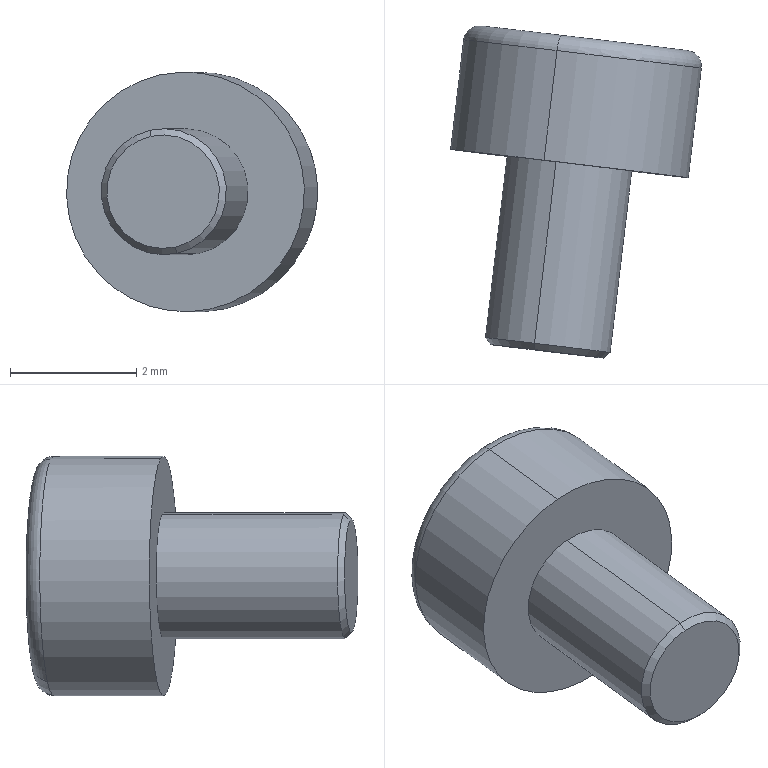Component | SolidWorks | hexagon socket head cap screws gb-2 | 1 solid | 25 faces | box 3.98 x 5.27 x 3.8 mm | volume 30 mm3 | plane 15 | cone 4 | cylinder 4 | torus 2 | commonest cylinder face diameters 2 x2 3.8 x2
STEP:
#1=CARTESIAN_POINT('',(-0.1815,3.084,0.2292));
#2=VERTEX_POINT('',#1);
#3=CARTESIAN_POINT('',(-0.1966,3.086,0.2984));
#4=VERTEX_POINT('',#3);
#5=CARTESIAN_POINT('',(-0.189,3.085,0.2638));
#6=DIRECTION('',(-0.1183,-0.993,0.001159));
#7=DIRECTION('',(0.2126,-0.02647,-0.9768));
#8=AXIS2_PLACEMENT_3D('',#5,#6,#7);
#9=CIRCLE('',#8,0.03543);
#10=EDGE_CURVE('',#2,#4,#9,.T.);
#11=ORIENTED_EDGE('',*,*,#10,.F.);
#12=CARTESIAN_POINT('',(-0.1802,3.088,0.2254));
#13=VERTEX_POINT('',#12);
#14=CARTESIAN_POINT('',(-0.1815,3.084,0.2292));
#15=DIRECTION('',(0.234,0.6834,-0.6915));
#16=VECTOR('',#15,39.37);
#17=LINE('',#14,#16);
#18=EDGE_CURVE('',#2,#13,#17,.T.);
#19=ORIENTED_EDGE('',*,*,#18,.T.);
#20=CARTESIAN_POINT('',(-0.1969,3.09,0.3023));
#21=VERTEX_POINT('',#20);
#22=CARTESIAN_POINT('',(-0.1886,3.089,0.2638));
#23=DIRECTION('',(0.1183,0.993,-0.001159));
#24=DIRECTION('',(0.2126,-0.02647,-0.9768));
#25=AXIS2_PLACEMENT_3D('',#22,#23,#24);
#26=CIRCLE('',#25,0.03937);
#27=EDGE_CURVE('',#21,#13,#26,.T.);
#28=ORIENTED_EDGE('',*,*,#27,.F.);
#29=CARTESIAN_POINT('',(-0.1966,3.086,0.2984));
#30=DIRECTION('',(-0.06668,0.7209,0.6899));
#31=VECTOR('',#30,39.37);
#32=LINE('',#29,#31);
#33=EDGE_CURVE('',#4,#21,#32,.T.);
#34=ORIENTED_EDGE('',*,*,#33,.F.);
#35=EDGE_LOOP('',(#11,#19,#28,#34));
#36=FACE_OUTER_BOUND('',#35,.T.);
#37=CARTESIAN_POINT('',(-0.189,3.085,0.2638));
#38=DIRECTION('',(0.1183,0.993,-0.001159));
#39=DIRECTION('',(-0.2126,0.02647,0.9768));
#40=AXIS2_PLACEMENT_3D('',#37,#38,#39);
#41=CONICAL_SURFACE('',#40,0.03543,0.7854);
#42=ADVANCED_FACE('',(#36),#41,.T.);
#43=CARTESIAN_POINT('',(-0.1796,3.283,0.3271));
#44=VERTEX_POINT('',#43);
#45=CARTESIAN_POINT('',(-0.1519,3.279,0.2002));
#46=VERTEX_POINT('',#45);
#47=CARTESIAN_POINT('',(-0.1658,3.281,0.2636));
#48=DIRECTION('',(0.1183,0.993,-0.001159));
#49=DIRECTION('',(0.2126,-0.02647,-0.9768));
#50=AXIS2_PLACEMENT_3D('',#47,#48,#49);
#51=CIRCLE('',#50,0.06496);
#52=EDGE_CURVE('',#44,#46,#51,.T.);
#53=ORIENTED_EDGE('',*,*,#52,.F.);
#54=CARTESIAN_POINT('',(-0.1828,3.273,0.3367));
#55=VERTEX_POINT('',#54);
#56=CARTESIAN_POINT('',(-0.1807,3.273,0.3271));
#57=DIRECTION('',(0.9699,-0.1153,0.2143));
#58=DIRECTION('',(0.2157,0.,-0.9765));
#59=AXIS2_PLACEMENT_3D('',#56,#57,#58);
#60=CIRCLE('',#59,0.009843);
#61=EDGE_CURVE('',#44,#55,#60,.T.);
#62=ORIENTED_EDGE('',*,*,#61,.T.);
#63=CARTESIAN_POINT('',(-0.151,3.269,0.1906));
#64=VERTEX_POINT('',#63);
#65=CARTESIAN_POINT('',(-0.1669,3.271,0.2636));
#66=DIRECTION('',(-0.1183,-0.993,0.001159));
#67=DIRECTION('',(0.2126,-0.02647,-0.9768));
#68=AXIS2_PLACEMENT_3D('',#65,#66,#67);
#69=CIRCLE('',#68,0.0748);
#70=EDGE_CURVE('',#64,#55,#69,.T.);
#71=ORIENTED_EDGE('',*,*,#70,.F.);
#72=CARTESIAN_POINT('',(-0.1531,3.269,0.2002));
#73=DIRECTION('',(-0.9699,0.1153,-0.2143));
#74=DIRECTION('',(-0.2157,0.,0.9765));
#75=AXIS2_PLACEMENT_3D('',#72,#73,#74);
#76=CIRCLE('',#75,0.009843);
#77=EDGE_CURVE('',#46,#64,#76,.T.);
#78=ORIENTED_EDGE('',*,*,#77,.F.);
#79=EDGE_LOOP('',(#53,#62,#71,#78));
#80=FACE_OUTER_BOUND('',#79,.T.);
#81=CARTESIAN_POINT('',(-0.1669,3.271,0.2636));
#82=DIRECTION('',(-0.1183,-0.993,0.001159));
#83=DIRECTION('',(0.2126,-0.02647,-0.9768));
#84=AXIS2_PLACEMENT_3D('',#81,#82,#83);
#85=TOROIDAL_SURFACE('',#84,0.06496,0.009843);
#86=ADVANCED_FACE('',(#80),#85,.T.);
#87=CARTESIAN_POINT('',(-0.1724,3.225,0.2637));
#88=VERTEX_POINT('',#87);
#89=CARTESIAN_POINT('',(-0.1767,3.243,0.2925));
#90=VERTEX_POINT('',#89);
#91=CARTESIAN_POINT('',(-0.1767,3.243,0.2925));
#92=DIRECTION('',(-0.125,0.5194,0.8453));
#93=VECTOR('',#92,39.37);
#94=LINE('',#91,#93);
#95=EDGE_CURVE('',#88,#90,#94,.T.);
#96=ORIENTED_EDGE('',*,*,#95,.F.);
#97=CARTESIAN_POINT('',(-0.1641,3.241,0.2348));
#98=VERTEX_POINT('',#97);
#99=CARTESIAN_POINT('',(-0.1641,3.241,0.2348));
#100=DIRECTION('',(0.2433,0.4736,-0.8465));
#101=VECTOR('',#100,39.37);
#102=LINE('',#99,#101);
#103=EDGE_CURVE('',#88,#98,#102,.T.);
#104=ORIENTED_EDGE('',*,*,#103,.T.);
#105=CARTESIAN_POINT('',(-0.1793,3.243,0.2355));
#106=VERTEX_POINT('',#105);
#107=CARTESIAN_POINT('',(-0.1704,3.242,0.2637));
#108=DIRECTION('',(-0.1183,-0.993,0.001159));
#109=DIRECTION('',(-0.2126,0.02647,0.9768));
#110=AXIS2_PLACEMENT_3D('',#107,#108,#109);
#111=CIRCLE('',#110,0.02953);
#112=EDGE_CURVE('',#106,#98,#111,.T.);
#113=ORIENTED_EDGE('',*,*,#112,.F.);
#114=CARTESIAN_POINT('',(-0.1991,3.245,0.2573));
#115=VERTEX_POINT('',#114);
#116=CARTESIAN_POINT('',(-0.1704,3.242,0.2637));
#117=DIRECTION('',(-0.1183,-0.993,0.001159));
#118=DIRECTION('',(-0.2126,0.02647,0.9768));
#119=AXIS2_PLACEMENT_3D('',#116,#117,#118);
#120=CIRCLE('',#119,0.02953);
#121=EDGE_CURVE('',#115,#106,#120,.T.);
#122=ORIENTED_EDGE('',*,*,#121,.F.);
#123=CARTESIAN_POINT('',(-0.1902,3.244,0.2855));
#124=VERTEX_POINT('',#123);
#125=CARTESIAN_POINT('',(-0.1704,3.242,0.2637));
#126=DIRECTION('',(-0.1183,-0.993,0.001159));
#127=DIRECTION('',(-0.2126,0.02647,0.9768));
#128=AXIS2_PLACEMENT_3D('',#125,#126,#127);
#129=CIRCLE('',#128,0.02953);
#130=EDGE_CURVE('',#124,#115,#129,.T.);
#131=ORIENTED_EDGE('',*,*,#130,.F.);
#132=CARTESIAN_POINT('',(-0.1704,3.242,0.2637));
#133=DIRECTION('',(-0.1183,-0.993,0.001159));
#134=DIRECTION('',(-0.2126,0.02647,0.9768));
#135=AXIS2_PLACEMENT_3D('',#132,#133,#134);
#136=CIRCLE('',#135,0.02953);
#137=EDGE_CURVE('',#90,#124,#136,.T.);
#138=ORIENTED_EDGE('',*,*,#137,.F.);
#139=EDGE_LOOP('',(#96,#104,#113,#122,#131,#138));
#140=FACE_OUTER_BOUND('',#139,.T.);
#141=CARTESIAN_POINT('',(-0.1704,3.242,0.2637));
#142=DIRECTION('',(0.1183,0.993,-0.001159));
#143=DIRECTION('',(-0.2126,0.02647,0.9768));
#144=AXIS2_PLACEMENT_3D('',#141,#142,#143);
#145=CONICAL_SURFACE('',#144,0.02953,1.047);
#146=ADVANCED_FACE('',(#140),#145,.F.);
#147=ORIENTED_EDGE('',*,*,#27,.T.);
#148=CARTESIAN_POINT('',(-0.1667,3.202,0.2252));
#149=VERTEX_POINT('',#148);
#150=CARTESIAN_POINT('',(-0.1807,3.084,0.2254));
#151=DIRECTION('',(0.1183,0.993,-0.001159));
#152=VECTOR('',#151,39.37);
#153=LINE('',#150,#152);
#154=EDGE_CURVE('',#13,#149,#153,.T.);
#155=ORIENTED_EDGE('',*,*,#154,.T.);
#156=CARTESIAN_POINT('',(-0.1834,3.204,0.3022));
#157=VERTEX_POINT('',#156);
#158=CARTESIAN_POINT('',(-0.1751,3.203,0.2637));
#159=DIRECTION('',(-0.1183,-0.993,0.001159));
#160=DIRECTION('',(0.2126,-0.02647,-0.9768));
#161=AXIS2_PLACEMENT_3D('',#158,#159,#160);
#162=CIRCLE('',#161,0.03937);
#163=EDGE_CURVE('',#149,#157,#162,.T.);
#164=ORIENTED_EDGE('',*,*,#163,.T.);
#165=CARTESIAN_POINT('',(-0.1974,3.086,0.3023));
#166=DIRECTION('',(0.1183,0.993,-0.001159));
#167=VECTOR('',#166,39.37);
#168=LINE('',#165,#167);
#169=EDGE_CURVE('',#21,#157,#168,.T.);
#170=ORIENTED_EDGE('',*,*,#169,.F.);
#171=EDGE_LOOP('',(#147,#155,#164,#170));
#172=FACE_OUTER_BOUND('',#171,.T.);
#173=CARTESIAN_POINT('',(-0.189,3.085,0.2638));
#174=DIRECTION('',(0.1183,0.993,-0.001159));
#175=DIRECTION('',(-0.2126,0.02647,0.9768));
#176=AXIS2_PLACEMENT_3D('',#173,#174,#175);
#177=CYLINDRICAL_SURFACE('',#176,0.03937);
#178=ADVANCED_FACE('',(#172),#177,.T.);
#179=CARTESIAN_POINT('',(-0.1592,3.201,0.1906));
#180=VERTEX_POINT('',#179);
#181=CARTESIAN_POINT('',(-0.191,3.205,0.3368));
#182=VERTEX_POINT('',#181);
#183=CARTESIAN_POINT('',(-0.1751,3.203,0.2637));
#184=DIRECTION('',(-0.1183,-0.993,0.001159));
#185=DIRECTION('',(0.2126,-0.02647,-0.9768));
#186=AXIS2_PLACEMENT_3D('',#183,#184,#185);
#187=CIRCLE('',#186,0.0748);
#188=EDGE_CURVE('',#180,#182,#187,.T.);
#189=ORIENTED_EDGE('',*,*,#188,.F.);
#190=CARTESIAN_POINT('',(-0.1592,3.201,0.1906));
#191=DIRECTION('',(0.1183,0.993,-0.001159));
#192=VECTOR('',#191,39.37);
#193=LINE('',#190,#192);
#194=EDGE_CURVE('',#180,#64,#193,.T.);
#195=ORIENTED_EDGE('',*,*,#194,.T.);
#196=ORIENTED_EDGE('',*,*,#70,.T.);
#197=CARTESIAN_POINT('',(-0.191,3.205,0.3368));
#198=DIRECTION('',(0.1183,0.993,-0.001159));
#199=VECTOR('',#198,39.37);
#200=LINE('',#197,#199);
#201=EDGE_CURVE('',#182,#55,#200,.T.);
#202=ORIENTED_EDGE('',*,*,#201,.F.);
#203=EDGE_LOOP('',(#189,#195,#196,#202));
#204=FACE_OUTER_BOUND('',#203,.T.);
#205=CARTESIAN_POINT('',(-0.1751,3.203,0.2637));
#206=DIRECTION('',(0.1183,0.993,-0.001159));
#207=DIRECTION('',(-0.2126,0.02647,0.9768));
#208=AXIS2_PLACEMENT_3D('',#205,#206,#207);
#209=CYLINDRICAL_SURFACE('',#208,0.0748);
#210=ADVANCED_FACE('',(#204),#209,.T.);
#211=CARTESIAN_POINT('',(-0.2027,3.246,0.274));
#212=VERTEX_POINT('',#211);
#213=CARTESIAN_POINT('',(-0.1777,3.243,0.297));
#214=DIRECTION('',(-0.7337,0.08664,-0.6739));
#215=VECTOR('',#214,39.37);
#216=LINE('',#213,#215);
#217=EDGE_CURVE('',#124,#212,#216,.T.);
#218=ORIENTED_EDGE('',*,*,#217,.F.);
#219=ORIENTED_EDGE('',*,*,#130,.T.);
#220=CARTESIAN_POINT('',(-0.2027,3.246,0.274));
#221=DIRECTION('',(0.2126,-0.02647,-0.9768));
#222=VECTOR('',#221,39.37);
#223=LINE('',#220,#222);
#224=EDGE_CURVE('',#212,#115,#223,.T.);
#225=ORIENTED_EDGE('',*,*,#224,.F.);
#226=EDGE_LOOP('',(#218,#219,#225));
#227=FACE_OUTER_BOUND('',#226,.T.);
#228=CARTESIAN_POINT('',(-0.2277,3.249,0.251));
#229=DIRECTION('',(0.1183,0.993,-0.001159));
#230=DIRECTION('',(-0.2126,0.02647,0.9768));
#231=AXIS2_PLACEMENT_3D('',#228,#229,#230);
#232=PLANE('',#231);
#233=ADVANCED_FACE('',(#227),#232,.T.);
#234=CARTESIAN_POINT('',(-0.1954,3.245,0.2407));
#235=VERTEX_POINT('',#234);
#236=CARTESIAN_POINT('',(-0.2027,3.246,0.274));
#237=DIRECTION('',(0.2126,-0.02647,-0.9768));
#238=VECTOR('',#237,39.37);
#239=LINE('',#236,#238);
#240=EDGE_CURVE('',#115,#235,#239,.T.);
#241=ORIENTED_EDGE('',*,*,#240,.F.);
#242=ORIENTED_EDGE('',*,*,#121,.T.);
#243=CARTESIAN_POINT('',(-0.1954,3.245,0.2407));
#244=DIRECTION('',(0.9463,-0.1131,-0.3028));
#245=VECTOR('',#244,39.37);
#246=LINE('',#243,#245);
#247=EDGE_CURVE('',#235,#106,#246,.T.);
#248=ORIENTED_EDGE('',*,*,#247,.F.);
#249=EDGE_LOOP('',(#241,#242,#248));
#250=FACE_OUTER_BOUND('',#249,.T.);
#251=CARTESIAN_POINT('',(-0.2277,3.249,0.251));
#252=DIRECTION('',(0.1183,0.993,-0.001159));
#253=DIRECTION('',(-0.2126,0.02647,0.9768));
#254=AXIS2_PLACEMENT_3D('',#251,#252,#253);
#255=PLANE('',#254);
#256=ADVANCED_FACE('',(#250),#255,.T.);
#257=CARTESIAN_POINT('',(-0.1632,3.241,0.2304));
#258=VERTEX_POINT('',#257);
#259=CARTESIAN_POINT('',(-0.1954,3.245,0.2407));
#260=DIRECTION('',(0.9463,-0.1131,-0.3028));
#261=VECTOR('',#260,39.37);
#262=LINE('',#259,#261);
#263=EDGE_CURVE('',#106,#258,#262,.T.);
#264=ORIENTED_EDGE('',*,*,#263,.F.);
#265=ORIENTED_EDGE('',*,*,#112,.T.);
#266=CARTESIAN_POINT('',(-0.1507,3.239,0.2418));
#267=VERTEX_POINT('',#266);
#268=CARTESIAN_POINT('',(-0.1704,3.242,0.2637));
#269=DIRECTION('',(-0.1183,-0.993,0.001159));
#270=DIRECTION('',(-0.2126,0.02647,0.9768));
#271=AXIS2_PLACEMENT_3D('',#268,#269,#270);
#272=CIRCLE('',#271,0.02953);
#273=EDGE_CURVE('',#98,#267,#272,.T.);
#274=ORIENTED_EDGE('',*,*,#273,.T.);
#275=CARTESIAN_POINT('',(-0.1632,3.241,0.2304));
#276=DIRECTION('',(0.7337,-0.08664,0.6739));
#277=VECTOR('',#276,39.37);
#278=LINE('',#275,#277);
#279=EDGE_CURVE('',#258,#267,#278,.T.);
#280=ORIENTED_EDGE('',*,*,#279,.F.);
#281=EDGE_LOOP('',(#264,#265,#274,#280));
#282=FACE_OUTER_BOUND('',#281,.T.);
#283=CARTESIAN_POINT('',(-0.2277,3.249,0.251));
#284=DIRECTION('',(0.1183,0.993,-0.001159));
#285=DIRECTION('',(-0.2126,0.02647,0.9768));
#286=AXIS2_PLACEMENT_3D('',#283,#284,#285);
#287=PLANE('',#286);
#288=ADVANCED_FACE('',(#282),#287,.T.);
#289=CARTESIAN_POINT('',(-0.1381,3.238,0.2533));
#290=VERTEX_POINT('',#289);
#291=CARTESIAN_POINT('',(-0.1632,3.241,0.2304));
#292=DIRECTION('',(0.7337,-0.08664,0.6739));
#293=VECTOR('',#292,39.37);
#294=LINE('',#291,#293);
#295=EDGE_CURVE('',#267,#290,#294,.T.);
#296=ORIENTED_EDGE('',*,*,#295,.F.);
#297=CARTESIAN_POINT('',(-0.1418,3.238,0.27));
#298=VERTEX_POINT('',#297);
#299=CARTESIAN_POINT('',(-0.1704,3.242,0.2637));
#300=DIRECTION('',(-0.1183,-0.993,0.001159));
#301=DIRECTION('',(0.2126,-0.02647,-0.9768));
#302=AXIS2_PLACEMENT_3D('',#299,#300,#301);
#303=CIRCLE('',#302,0.02953);
#304=EDGE_CURVE('',#267,#298,#303,.T.);
#305=ORIENTED_EDGE('',*,*,#304,.T.);
#306=CARTESIAN_POINT('',(-0.1381,3.238,0.2533));
#307=DIRECTION('',(-0.2126,0.02647,0.9768));
#308=VECTOR('',#307,39.37);
#309=LINE('',#306,#308);
#310=EDGE_CURVE('',#290,#298,#309,.T.);
#311=ORIENTED_EDGE('',*,*,#310,.F.);
#312=EDGE_LOOP('',(#296,#305,#311));
#313=FACE_OUTER_BOUND('',#312,.T.);
#314=CARTESIAN_POINT('',(-0.2277,3.249,0.251));
#315=DIRECTION('',(0.1183,0.993,-0.001159));
#316=DIRECTION('',(-0.2126,0.02647,0.9768));
#317=AXIS2_PLACEMENT_3D('',#314,#315,#316);
#318=PLANE('',#317);
#319=ADVANCED_FACE('',(#313),#318,.T.);
#320=CARTESIAN_POINT('',(-0.1454,3.239,0.2866));
#321=VERTEX_POINT('',#320);
#322=CARTESIAN_POINT('',(-0.1381,3.238,0.2533));
#323=DIRECTION('',(-0.2126,0.02647,0.9768));
#324=VECTOR('',#323,39.37);
#325=LINE('',#322,#324);
#326=EDGE_CURVE('',#298,#321,#325,.T.);
#327=ORIENTED_EDGE('',*,*,#326,.F.);
#328=CARTESIAN_POINT('',(-0.1615,3.241,0.2918));
#329=VERTEX_POINT('',#328);
#330=CARTESIAN_POINT('',(-0.1704,3.242,0.2637));
#331=DIRECTION('',(-0.1183,-0.993,0.001159));
#332=DIRECTION('',(-0.2126,0.02647,0.9768));
#333=AXIS2_PLACEMENT_3D('',#330,#331,#332);
#334=CIRCLE('',#333,0.02953);
#335=EDGE_CURVE('',#298,#329,#334,.T.);
#336=ORIENTED_EDGE('',*,*,#335,.T.);
#337=CARTESIAN_POINT('',(-0.1454,3.239,0.2866));
#338=DIRECTION('',(-0.9463,0.1131,0.3028));
#339=VECTOR('',#338,39.37);
#340=LINE('',#337,#339);
#341=EDGE_CURVE('',#321,#329,#340,.T.);
#342=ORIENTED_EDGE('',*,*,#341,.F.);
#343=EDGE_LOOP('',(#327,#336,#342));
#344=FACE_OUTER_BOUND('',#343,.T.);
#345=CARTESIAN_POINT('',(-0.2277,3.249,0.251));
#346=DIRECTION('',(0.1183,0.993,-0.001159));
#347=DIRECTION('',(-0.2126,0.02647,0.9768));
#348=AXIS2_PLACEMENT_3D('',#345,#346,#347);
#349=PLANE('',#348);
#350=ADVANCED_FACE('',(#344),#349,.T.);
#351=CARTESIAN_POINT('',(-0.1777,3.243,0.297));
#352=VERTEX_POINT('',#351);
#353=CARTESIAN_POINT('',(-0.1454,3.239,0.2866));
#354=DIRECTION('',(-0.9463,0.1131,0.3028));
#355=VECTOR('',#354,39.37);
#356=LINE('',#353,#355);
#357=EDGE_CURVE('',#329,#352,#356,.T.);
#358=ORIENTED_EDGE('',*,*,#357,.F.);
#359=CARTESIAN_POINT('',(-0.1704,3.242,0.2637));
#360=DIRECTION('',(-0.1183,-0.993,0.001159));
#361=DIRECTION('',(-0.2126,0.02647,0.9768));
#362=AXIS2_PLACEMENT_3D('',#359,#360,#361);
#363=CIRCLE('',#362,0.02953);
#364=EDGE_CURVE('',#329,#90,#363,.T.);
#365=ORIENTED_EDGE('',*,*,#364,.T.);
#366=ORIENTED_EDGE('',*,*,#137,.T.);
#367=CARTESIAN_POINT('',(-0.1777,3.243,0.297));
#368=DIRECTION('',(-0.7337,0.08664,-0.6739));
#369=VECTOR('',#368,39.37);
#370=LINE('',#367,#369);
#371=EDGE_CURVE('',#352,#124,#370,.T.);
#372=ORIENTED_EDGE('',*,*,#371,.F.);
#373=EDGE_LOOP('',(#358,#365,#366,#372));
#374=FACE_OUTER_BOUND('',#373,.T.);
#375=CARTESIAN_POINT('',(-0.2277,3.249,0.251));
#376=DIRECTION('',(0.1183,0.993,-0.001159));
#377=DIRECTION('',(-0.2126,0.02647,0.9768));
#378=AXIS2_PLACEMENT_3D('',#375,#376,#377);
#379=PLANE('',#378);
#380=ADVANCED_FACE('',(#374),#379,.T.);
#381=CARTESIAN_POINT('',(-0.1658,3.281,0.2636));
#382=DIRECTION('',(0.1183,0.993,-0.001159));
#383=DIRECTION('',(0.2126,-0.02647,-0.9768));
#384=AXIS2_PLACEMENT_3D('',#381,#382,#383);
#385=CIRCLE('',#384,0.06496);
#386=EDGE_CURVE('',#46,#44,#385,.T.);
#387=ORIENTED_EDGE('',*,*,#386,.T.);
#388=ORIENTED_EDGE('',*,*,#52,.T.);
#389=EDGE_LOOP('',(#387,#388));
#390=FACE_OUTER_BOUND('',#389,.T.);
#391=CARTESIAN_POINT('',(-0.1908,3.284,0.2406));
#392=VERTEX_POINT('',#391);
#393=CARTESIAN_POINT('',(-0.1585,3.28,0.2303));
#394=VERTEX_POINT('',#393);
#395=CARTESIAN_POINT('',(-0.1908,3.284,0.2406));
#396=DIRECTION('',(0.9463,-0.1131,-0.3028));
#397=VECTOR('',#396,39.37);
#398=LINE('',#395,#397);
#399=EDGE_CURVE('',#392,#394,#398,.T.);
#400=ORIENTED_EDGE('',*,*,#399,.T.);
#401=CARTESIAN_POINT('',(-0.1335,3.277,0.2533));
#402=VERTEX_POINT('',#401);
#403=CARTESIAN_POINT('',(-0.1585,3.28,0.2303));
#404=DIRECTION('',(0.7337,-0.08664,0.6739));
#405=VECTOR('',#404,39.37);
#406=LINE('',#403,#405);
#407=EDGE_CURVE('',#394,#402,#406,.T.);
#408=ORIENTED_EDGE('',*,*,#407,.T.);
#409=CARTESIAN_POINT('',(-0.1407,3.278,0.2866));
#410=VERTEX_POINT('',#409);
#411=CARTESIAN_POINT('',(-0.1335,3.277,0.2533));
#412=DIRECTION('',(-0.2126,0.02647,0.9768));
#413=VECTOR('',#412,39.37);
#414=LINE('',#411,#413);
#415=EDGE_CURVE('',#402,#410,#414,.T.);
#416=ORIENTED_EDGE('',*,*,#415,.T.);
#417=CARTESIAN_POINT('',(-0.173,3.282,0.2969));
#418=VERTEX_POINT('',#417);
#419=CARTESIAN_POINT('',(-0.1407,3.278,0.2866));
#420=DIRECTION('',(-0.9463,0.1131,0.3028));
#421=VECTOR('',#420,39.37);
#422=LINE('',#419,#421);
#423=EDGE_CURVE('',#410,#418,#422,.T.);
#424=ORIENTED_EDGE('',*,*,#423,.T.);
#425=CARTESIAN_POINT('',(-0.198,3.285,0.2739));
#426=VERTEX_POINT('',#425);
#427=CARTESIAN_POINT('',(-0.173,3.282,0.2969));
#428=DIRECTION('',(-0.7337,0.08664,-0.6739));
#429=VECTOR('',#428,39.37);
#430=LINE('',#427,#429);
#431=EDGE_CURVE('',#418,#426,#430,.T.);
#432=ORIENTED_EDGE('',*,*,#431,.T.);
#433=CARTESIAN_POINT('',(-0.198,3.285,0.2739));
#434=DIRECTION('',(0.2126,-0.02647,-0.9768));
#435=VECTOR('',#434,39.37);
#436=LINE('',#433,#435);
#437=EDGE_CURVE('',#426,#392,#436,.T.);
#438=ORIENTED_EDGE('',*,*,#437,.T.);
#439=EDGE_LOOP('',(#400,#408,#416,#424,#432,#438));
#440=FACE_BOUND('',#439,.T.);
#441=CARTESIAN_POINT('',(-0.1658,3.281,0.2636));
#442=DIRECTION('',(-0.1183,-0.993,0.001159));
#443=DIRECTION('',(0.2126,-0.02647,-0.9768));
#444=AXIS2_PLACEMENT_3D('',#441,#442,#443);
#445=PLANE('',#444);
#446=ADVANCED_FACE('',(#390,#440),#445,.F.);
#447=CARTESIAN_POINT('',(-0.1751,3.203,0.2637));
#448=DIRECTION('',(-0.1183,-0.993,0.001159));
#449=DIRECTION('',(0.2126,-0.02647,-0.9768));
#450=AXIS2_PLACEMENT_3D('',#447,#448,#449);
#451=CIRCLE('',#450,0.0748);
#452=EDGE_CURVE('',#182,#180,#451,.T.);
#453=ORIENTED_EDGE('',*,*,#452,.T.);
#454=ORIENTED_EDGE('',*,*,#188,.T.);
#455=EDGE_LOOP('',(#453,#454));
#456=FACE_OUTER_BOUND('',#455,.T.);
#457=CARTESIAN_POINT('',(-0.1751,3.203,0.2637));
#458=DIRECTION('',(-0.1183,-0.993,0.001159));
#459=DIRECTION('',(0.2126,-0.02647,-0.9768));
#460=AXIS2_PLACEMENT_3D('',#457,#458,#459);
#461=CIRCLE('',#460,0.03937);
#462=EDGE_CURVE('',#157,#149,#461,.T.);
#463=ORIENTED_EDGE('',*,*,#462,.F.);
#464=ORIENTED_EDGE('',*,*,#163,.F.);
#465=EDGE_LOOP('',(#463,#464));
#466=FACE_BOUND('',#465,.T.);
#467=CARTESIAN_POINT('',(-0.1751,3.203,0.2637));
#468=DIRECTION('',(-0.1183,-0.993,0.001159));
#469=DIRECTION('',(0.2126,-0.02647,-0.9768));
#470=AXIS2_PLACEMENT_3D('',#467,#468,#469);
#471=PLANE('',#470);
#472=ADVANCED_FACE('',(#456,#466),#471,.T.);
#473=ORIENTED_EDGE('',*,*,#194,.F.);
#474=ORIENTED_EDGE('',*,*,#452,.F.);
#475=ORIENTED_EDGE('',*,*,#201,.T.);
#476=CARTESIAN_POINT('',(-0.1669,3.271,0.2636));
#477=DIRECTION('',(-0.1183,-0.993,0.001159));
#478=DIRECTION('',(0.2126,-0.02647,-0.9768));
#479=AXIS2_PLACEMENT_3D('',#476,#477,#478);
#480=CIRCLE('',#479,0.0748);
#481=EDGE_CURVE('',#55,#64,#480,.T.);
#482=ORIENTED_EDGE('',*,*,#481,.T.);
#483=EDGE_LOOP('',(#473,#474,#475,#482));
#484=FACE_OUTER_BOUND('',#483,.T.);
#485=CARTESIAN_POINT('',(-0.1751,3.203,0.2637));
#486=DIRECTION('',(0.1183,0.993,-0.001159));
#487=DIRECTION('',(-0.2126,0.02647,0.9768));
#488=AXIS2_PLACEMENT_3D('',#485,#486,#487);
#489=CYLINDRICAL_SURFACE('',#488,0.0748);
#490=ADVANCED_FACE('',(#484),#489,.T.);
#491=ORIENTED_EDGE('',*,*,#154,.F.);
#492=CARTESIAN_POINT('',(-0.1886,3.089,0.2638));
#493=DIRECTION('',(0.1183,0.993,-0.001159));
#494=DIRECTION('',(0.2126,-0.02647,-0.9768));
#495=AXIS2_PLACEMENT_3D('',#492,#493,#494);
#496=CIRCLE('',#495,0.03937);
#497=EDGE_CURVE('',#13,#21,#496,.T.);
#498=ORIENTED_EDGE('',*,*,#497,.T.);
#499=ORIENTED_EDGE('',*,*,#169,.T.);
#500=ORIENTED_EDGE('',*,*,#462,.T.);
#501=EDGE_LOOP('',(#491,#498,#499,#500));
#502=FACE_OUTER_BOUND('',#501,.T.);
#503=CARTESIAN_POINT('',(-0.189,3.085,0.2638));
#504=DIRECTION('',(0.1183,0.993,-0.001159));
#505=DIRECTION('',(-0.2126,0.02647,0.9768));
#506=AXIS2_PLACEMENT_3D('',#503,#504,#505);
#507=CYLINDRICAL_SURFACE('',#506,0.03937);
#508=ADVANCED_FACE('',(#502),#507,.T.);
#509=CARTESIAN_POINT('',(-0.189,3.085,0.2638));
#510=DIRECTION('',(-0.1183,-0.993,0.001159));
#511=DIRECTION('',(0.2126,-0.02647,-0.9768));
#512=AXIS2_PLACEMENT_3D('',#509,#510,#511);
#513=CIRCLE('',#512,0.03543);
#514=EDGE_CURVE('',#4,#2,#513,.T.);
#515=ORIENTED_EDGE('',*,*,#514,.T.);
#516=ORIENTED_EDGE('',*,*,#10,.T.);
#517=EDGE_LOOP('',(#515,#516));
#518=FACE_OUTER_BOUND('',#517,.T.);
#519=CARTESIAN_POINT('',(-0.189,3.085,0.2638));
#520=DIRECTION('',(-0.1183,-0.993,0.001159));
#521=DIRECTION('',(0.2126,-0.02647,-0.9768));
#522=AXIS2_PLACEMENT_3D('',#519,#520,#521);
#523=PLANE('',#522);
#524=ADVANCED_FACE('',(#518),#523,.T.);
#525=ORIENTED_EDGE('',*,*,#399,.F.);
#526=CARTESIAN_POINT('',(-0.1954,3.245,0.2407));
#527=DIRECTION('',(0.1183,0.993,-0.001159));
#528=VECTOR('',#527,39.37);
#529=LINE('',#526,#528);
#530=EDGE_CURVE('',#235,#392,#529,.T.);
#531=ORIENTED_EDGE('',*,*,#530,.F.);
#532=ORIENTED_EDGE('',*,*,#247,.T.);
#533=ORIENTED_EDGE('',*,*,#263,.T.);
#534=CARTESIAN_POINT('',(-0.1632,3.241,0.2304));
#535=DIRECTION('',(0.1183,0.993,-0.001159));
#536=VECTOR('',#535,39.37);
#537=LINE('',#534,#536);
#538=EDGE_CURVE('',#258,#394,#537,.T.);
#539=ORIENTED_EDGE('',*,*,#538,.T.);
#540=EDGE_LOOP('',(#525,#531,#532,#533,#539));
#541=FACE_OUTER_BOUND('',#540,.T.);
#542=CARTESIAN_POINT('',(-0.1954,3.245,0.2407));
#543=DIRECTION('',(0.3008,-0.03474,0.953));
#544=DIRECTION('',(-0.9463,0.1131,0.3028));
#545=AXIS2_PLACEMENT_3D('',#542,#543,#544);
#546=PLANE('',#545);
#547=ADVANCED_FACE('',(#541),#546,.T.);
#548=ORIENTED_EDGE('',*,*,#407,.F.);
#549=ORIENTED_EDGE('',*,*,#538,.F.);
#550=ORIENTED_EDGE('',*,*,#279,.T.);
#551=ORIENTED_EDGE('',*,*,#295,.T.);
#552=CARTESIAN_POINT('',(-0.1381,3.238,0.2533));
#553=DIRECTION('',(0.1183,0.993,-0.001159));
#554=VECTOR('',#553,39.37);
#555=LINE('',#552,#554);
#556=EDGE_CURVE('',#290,#402,#555,.T.);
#557=ORIENTED_EDGE('',*,*,#556,.T.);
#558=EDGE_LOOP('',(#548,#549,#550,#551,#557));
#559=FACE_OUTER_BOUND('',#558,.T.);
#560=CARTESIAN_POINT('',(-0.1632,3.241,0.2304));
#561=DIRECTION('',(-0.6691,0.08059,0.7388));
#562=DIRECTION('',(-0.7337,0.08664,-0.6739));
#563=AXIS2_PLACEMENT_3D('',#560,#561,#562);
#564=PLANE('',#563);
#565=ADVANCED_FACE('',(#559),#564,.T.);
#566=ORIENTED_EDGE('',*,*,#415,.F.);
#567=ORIENTED_EDGE('',*,*,#556,.F.);
#568=ORIENTED_EDGE('',*,*,#310,.T.);
#569=ORIENTED_EDGE('',*,*,#326,.T.);
#570=CARTESIAN_POINT('',(-0.1454,3.239,0.2866));
#571=DIRECTION('',(0.1183,0.993,-0.001159));
#572=VECTOR('',#571,39.37);
#573=LINE('',#570,#572);
#574=EDGE_CURVE('',#321,#410,#573,.T.);
#575=ORIENTED_EDGE('',*,*,#574,.T.);
#576=EDGE_LOOP('',(#566,#567,#568,#569,#575));
#577=FACE_OUTER_BOUND('',#576,.T.);
#578=CARTESIAN_POINT('',(-0.1381,3.238,0.2533));
#579=DIRECTION('',(-0.9699,0.1153,-0.2143));
#580=DIRECTION('',(0.2126,-0.02647,-0.9768));
#581=AXIS2_PLACEMENT_3D('',#578,#579,#580);
#582=PLANE('',#581);
#583=ADVANCED_FACE('',(#577),#582,.T.);
#584=ORIENTED_EDGE('',*,*,#423,.F.);
#585=ORIENTED_EDGE('',*,*,#574,.F.);
#586=ORIENTED_EDGE('',*,*,#341,.T.);
#587=ORIENTED_EDGE('',*,*,#357,.T.);
#588=CARTESIAN_POINT('',(-0.1777,3.243,0.297));
#589=DIRECTION('',(0.1183,0.993,-0.001159));
#590=VECTOR('',#589,39.37);
#591=LINE('',#588,#590);
#592=EDGE_CURVE('',#352,#418,#591,.T.);
#593=ORIENTED_EDGE('',*,*,#592,.T.);
#594=EDGE_LOOP('',(#584,#585,#586,#587,#593));
#595=FACE_OUTER_BOUND('',#594,.T.);
#596=CARTESIAN_POINT('',(-0.1454,3.239,0.2866));
#597=DIRECTION('',(-0.3008,0.03474,-0.953));
#598=DIRECTION('',(0.9463,-0.1131,-0.3028));
#599=AXIS2_PLACEMENT_3D('',#596,#597,#598);
#600=PLANE('',#599);
#601=ADVANCED_FACE('',(#595),#600,.T.);
#602=ORIENTED_EDGE('',*,*,#431,.F.);
#603=ORIENTED_EDGE('',*,*,#592,.F.);
#604=ORIENTED_EDGE('',*,*,#371,.T.);
#605=ORIENTED_EDGE('',*,*,#217,.T.);
#606=CARTESIAN_POINT('',(-0.2027,3.246,0.274));
#607=DIRECTION('',(0.1183,0.993,-0.001159));
#608=VECTOR('',#607,39.37);
#609=LINE('',#606,#608);
#610=EDGE_CURVE('',#212,#426,#609,.T.);
#611=ORIENTED_EDGE('',*,*,#610,.T.);
#612=EDGE_LOOP('',(#602,#603,#604,#605,#611));
#613=FACE_OUTER_BOUND('',#612,.T.);
#614=CARTESIAN_POINT('',(-0.1777,3.243,0.297));
#615=DIRECTION('',(0.6691,-0.08059,-0.7388));
#616=DIRECTION('',(0.7337,-0.08664,0.6739));
#617=AXIS2_PLACEMENT_3D('',#614,#615,#616);
#618=PLANE('',#617);
#619=ADVANCED_FACE('',(#613),#618,.T.);
#620=ORIENTED_EDGE('',*,*,#437,.F.);
#621=ORIENTED_EDGE('',*,*,#610,.F.);
#622=ORIENTED_EDGE('',*,*,#224,.T.);
#623=ORIENTED_EDGE('',*,*,#240,.T.);
#624=ORIENTED_EDGE('',*,*,#530,.T.);
#625=EDGE_LOOP('',(#620,#621,#622,#623,#624));
#626=FACE_OUTER_BOUND('',#625,.T.);
#627=CARTESIAN_POINT('',(-0.2027,3.246,0.274));
#628=DIRECTION('',(0.9699,-0.1153,0.2143));
#629=DIRECTION('',(-0.2126,0.02647,0.9768));
#630=AXIS2_PLACEMENT_3D('',#627,#628,#629);
#631=PLANE('',#630);
#632=ADVANCED_FACE('',(#626),#631,.T.);
#633=ORIENTED_EDGE('',*,*,#103,.F.);
#634=ORIENTED_EDGE('',*,*,#95,.T.);
#635=ORIENTED_EDGE('',*,*,#364,.F.);
#636=ORIENTED_EDGE('',*,*,#335,.F.);
#637=ORIENTED_EDGE('',*,*,#304,.F.);
#638=ORIENTED_EDGE('',*,*,#273,.F.);
#639=EDGE_LOOP('',(#633,#634,#635,#636,#637,#638));
#640=FACE_OUTER_BOUND('',#639,.T.);
#641=CARTESIAN_POINT('',(-0.1704,3.242,0.2637));
#642=DIRECTION('',(0.1183,0.993,-0.001159));
#643=DIRECTION('',(-0.2126,0.02647,0.9768));
#644=AXIS2_PLACEMENT_3D('',#641,#642,#643);
#645=CONICAL_SURFACE('',#644,0.02953,1.047);
#646=ADVANCED_FACE('',(#640),#645,.F.);
#647=ORIENTED_EDGE('',*,*,#61,.F.);
#648=ORIENTED_EDGE('',*,*,#386,.F.);
#649=ORIENTED_EDGE('',*,*,#77,.T.);
#650=ORIENTED_EDGE('',*,*,#481,.F.);
#651=EDGE_LOOP('',(#647,#648,#649,#650));
#652=FACE_OUTER_BOUND('',#651,.T.);
#653=CARTESIAN_POINT('',(-0.1669,3.271,0.2636));
#654=DIRECTION('',(-0.1183,-0.993,0.001159));
#655=DIRECTION('',(0.2126,-0.02647,-0.9768));
#656=AXIS2_PLACEMENT_3D('',#653,#654,#655);
#657=TOROIDAL_SURFACE('',#656,0.06496,0.009843);
#658=ADVANCED_FACE('',(#652),#657,.T.);
#659=ORIENTED_EDGE('',*,*,#18,.F.);
#660=ORIENTED_EDGE('',*,*,#514,.F.);
#661=ORIENTED_EDGE('',*,*,#33,.T.);
#662=ORIENTED_EDGE('',*,*,#497,.F.);
#663=EDGE_LOOP('',(#659,#660,#661,#662));
#664=FACE_OUTER_BOUND('',#663,.T.);
#665=CARTESIAN_POINT('',(-0.189,3.085,0.2638));
#666=DIRECTION('',(0.1183,0.993,-0.001159));
#667=DIRECTION('',(-0.2126,0.02647,0.9768));
#668=AXIS2_PLACEMENT_3D('',#665,#666,#667);
#669=CONICAL_SURFACE('',#668,0.03543,0.7854);
#670=ADVANCED_FACE('',(#664),#669,.T.);
#671=CLOSED_SHELL('',(#42,#86,#146,#178,#210,#233,#256,#288,#319,#350,#380,#446,#472,#490,#508,#524,#547,#565,#583,#601,#619,#632,#646,#658,#670));
#672=MANIFOLD_SOLID_BREP('',#671);
#673=CARTESIAN_POINT('',(0.,0.,0.));
#674=DIRECTION('',(0.,0.,1.));
#675=DIRECTION('',(1.,0.,0.));
#676=AXIS2_PLACEMENT_3D('',#673,#674,#675);
#677=(LENGTH_UNIT()NAMED_UNIT(*)SI_UNIT($,.METRE.));
#678=LENGTH_MEASURE_WITH_UNIT(LENGTH_MEASURE(0.0254),#677);
#679=DIMENSIONAL_EXPONENTS(1.,0.,0.,0.,0.,0.,0.);
#680=(CONVERSION_BASED_UNIT('',#678)LENGTH_UNIT()NAMED_UNIT(#679));
#681=UNCERTAINTY_MEASURE_WITH_UNIT(LENGTH_MEASURE(0.00001),#680,'','');
#682=(NAMED_UNIT(*)PLANE_ANGLE_UNIT()SI_UNIT($,.RADIAN.));
#683=(NAMED_UNIT(*)SI_UNIT($,.STERADIAN.)SOLID_ANGLE_UNIT());
#684=(GEOMETRIC_REPRESENTATION_CONTEXT(3)GLOBAL_UNCERTAINTY_ASSIGNED_CONTEXT((#681))GLOBAL_UNIT_ASSIGNED_CONTEXT((#680,#682,#683))REPRESENTATION_CONTEXT('',''));
#685=ADVANCED_BREP_SHAPE_REPRESENTATION('',(#672,#676),#684);
#686=COLOUR_RGB('',0.7922,0.8196,0.9333);
#687=FILL_AREA_STYLE_COLOUR('',#686);
#688=FILL_AREA_STYLE('',(#687));
#689=SURFACE_STYLE_FILL_AREA(#688);
#690=SURFACE_SIDE_STYLE('',(#689));
#691=SURFACE_STYLE_USAGE(.BOTH.,#690);
#692=PRESENTATION_STYLE_ASSIGNMENT((#691));
#693=STYLED_ITEM('',(#692),#672);
#694=PRESENTATION_LAYER_ASSIGNMENT('','',(#693));
#695=(LENGTH_UNIT()NAMED_UNIT(*)SI_UNIT($,.METRE.));
#696=LENGTH_MEASURE_WITH_UNIT(LENGTH_MEASURE(0.0254),#695);
#697=DIMENSIONAL_EXPONENTS(1.,0.,0.,0.,0.,0.,0.);
#698=(CONVERSION_BASED_UNIT('',#696)LENGTH_UNIT()NAMED_UNIT(#697));
#699=UNCERTAINTY_MEASURE_WITH_UNIT(LENGTH_MEASURE(0.00001),#698,'','');
#700=(NAMED_UNIT(*)PLANE_ANGLE_UNIT()SI_UNIT($,.RADIAN.));
#701=(NAMED_UNIT(*)SI_UNIT($,.STERADIAN.)SOLID_ANGLE_UNIT());
#702=(GEOMETRIC_REPRESENTATION_CONTEXT(3)GLOBAL_UNCERTAINTY_ASSIGNED_CONTEXT((#699))GLOBAL_UNIT_ASSIGNED_CONTEXT((#698,#700,#701))REPRESENTATION_CONTEXT('',''));
#703=MECHANICAL_DESIGN_GEOMETRIC_PRESENTATION_REPRESENTATION('',(#693),#702);